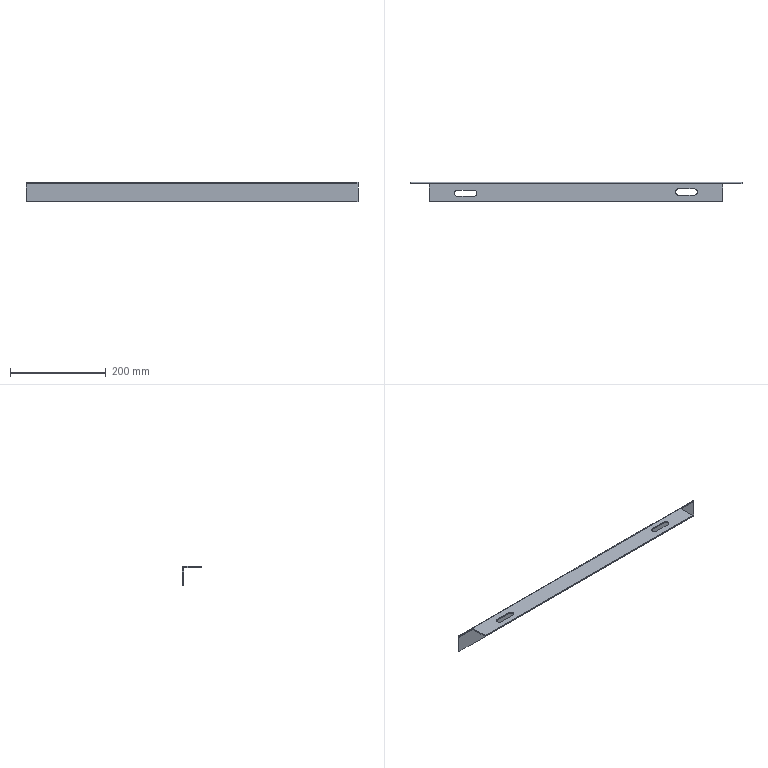Component | SolidWorks | BottomFrameAssembly2-1_CabinetWidthBeam-1 | 1 solid | 27 faces | box 695 x 40 x 40 mm | volume 123113 mm3 | plane 19 | cylinder 8 | commonest cylinder face diameters 13 x6 1 x1 6 x1
STEP:
#1=COLOUR_RGB('',0.7922,0.8196,0.9333);
#2=FILL_AREA_STYLE_COLOUR('',#1);
#3=FILL_AREA_STYLE('',(#2));
#4=SURFACE_STYLE_FILL_AREA(#3);
#5=SURFACE_SIDE_STYLE('',(#4));
#6=SURFACE_STYLE_USAGE(.BOTH.,#5);
#7=PRESENTATION_STYLE_ASSIGNMENT((#6));
#8=CARTESIAN_POINT('',(-1.991,5.157,66.928));
#9=VERTEX_POINT('',#8);
#10=CARTESIAN_POINT('',(-1.735,5.413,66.928));
#11=VERTEX_POINT('',#10);
#12=CARTESIAN_POINT('',(-1.735,5.157,66.928));
#13=DIRECTION('',(0.,-0.,-1.));
#14=DIRECTION('',(-1.,-0.,0.));
#15=AXIS2_PLACEMENT_3D('',#12,#13,#14);
#16=CIRCLE('',#15,0.2559);
#17=EDGE_CURVE('',#9,#11,#16,.T.);
#18=ORIENTED_EDGE('',*,*,#17,.F.);
#19=CARTESIAN_POINT('',(-1.991,5.157,66.83));
#20=VERTEX_POINT('',#19);
#21=CARTESIAN_POINT('',(-1.991,5.157,66.928));
#22=DIRECTION('',(0.,-0.,-1.));
#23=VECTOR('',#22,39.37);
#24=LINE('',#21,#23);
#25=EDGE_CURVE('',#9,#20,#24,.T.);
#26=ORIENTED_EDGE('',*,*,#25,.T.);
#27=CARTESIAN_POINT('',(-1.735,5.413,66.83));
#28=VERTEX_POINT('',#27);
#29=CARTESIAN_POINT('',(-1.735,5.157,66.83));
#30=DIRECTION('',(0.,-0.,-1.));
#31=DIRECTION('',(-1.,-0.,0.));
#32=AXIS2_PLACEMENT_3D('',#29,#30,#31);
#33=CIRCLE('',#32,0.2559);
#34=EDGE_CURVE('',#20,#28,#33,.T.);
#35=ORIENTED_EDGE('',*,*,#34,.T.);
#36=CARTESIAN_POINT('',(-1.735,5.413,66.928));
#37=DIRECTION('',(0.,-0.,-1.));
#38=VECTOR('',#37,39.37);
#39=LINE('',#36,#38);
#40=EDGE_CURVE('',#11,#28,#39,.T.);
#41=ORIENTED_EDGE('',*,*,#40,.F.);
#42=EDGE_LOOP('',(#18,#26,#35,#41));
#43=FACE_OUTER_BOUND('',#42,.T.);
#44=CARTESIAN_POINT('',(-1.735,5.157,66.928));
#45=DIRECTION('',(0.,-0.,-1.));
#46=DIRECTION('',(-1.,-0.,0.));
#47=AXIS2_PLACEMENT_3D('',#44,#45,#46);
#48=CYLINDRICAL_SURFACE('',#47,0.2559);
#49=ADVANCED_FACE('',(#43),#48,.F.);
#50=CARTESIAN_POINT('',(16.198,5.265,66.928));
#51=VERTEX_POINT('',#50);
#52=CARTESIAN_POINT('',(16.454,5.521,66.928));
#53=VERTEX_POINT('',#52);
#54=CARTESIAN_POINT('',(16.454,5.265,66.928));
#55=DIRECTION('',(0.,-0.,-1.));
#56=DIRECTION('',(-1.,-0.,0.));
#57=AXIS2_PLACEMENT_3D('',#54,#55,#56);
#58=CIRCLE('',#57,0.2559);
#59=EDGE_CURVE('',#51,#53,#58,.T.);
#60=ORIENTED_EDGE('',*,*,#59,.F.);
#61=CARTESIAN_POINT('',(16.198,5.265,66.83));
#62=VERTEX_POINT('',#61);
#63=CARTESIAN_POINT('',(16.198,5.265,66.928));
#64=DIRECTION('',(0.,-0.,-1.));
#65=VECTOR('',#64,39.37);
#66=LINE('',#63,#65);
#67=EDGE_CURVE('',#51,#62,#66,.T.);
#68=ORIENTED_EDGE('',*,*,#67,.T.);
#69=CARTESIAN_POINT('',(16.454,5.521,66.83));
#70=VERTEX_POINT('',#69);
#71=CARTESIAN_POINT('',(16.454,5.265,66.83));
#72=DIRECTION('',(0.,-0.,-1.));
#73=DIRECTION('',(-1.,-0.,0.));
#74=AXIS2_PLACEMENT_3D('',#71,#72,#73);
#75=CIRCLE('',#74,0.2559);
#76=EDGE_CURVE('',#62,#70,#75,.T.);
#77=ORIENTED_EDGE('',*,*,#76,.T.);
#78=CARTESIAN_POINT('',(16.454,5.521,66.928));
#79=DIRECTION('',(0.,-0.,-1.));
#80=VECTOR('',#79,39.37);
#81=LINE('',#78,#80);
#82=EDGE_CURVE('',#53,#70,#81,.T.);
#83=ORIENTED_EDGE('',*,*,#82,.F.);
#84=EDGE_LOOP('',(#60,#68,#77,#83));
#85=FACE_OUTER_BOUND('',#84,.T.);
#86=CARTESIAN_POINT('',(16.454,5.265,66.928));
#87=DIRECTION('',(0.,-0.,-1.));
#88=DIRECTION('',(-1.,-0.,0.));
#89=AXIS2_PLACEMENT_3D('',#86,#87,#88);
#90=CYLINDRICAL_SURFACE('',#89,0.2559);
#91=ADVANCED_FACE('',(#85),#90,.F.);
#92=CARTESIAN_POINT('',(-0.4356,5.413,66.83));
#93=VERTEX_POINT('',#92);
#94=CARTESIAN_POINT('',(-0.4356,4.901,66.83));
#95=VERTEX_POINT('',#94);
#96=CARTESIAN_POINT('',(-0.4356,5.157,66.83));
#97=DIRECTION('',(0.,-0.,-1.));
#98=DIRECTION('',(-1.,-0.,0.));
#99=AXIS2_PLACEMENT_3D('',#96,#97,#98);
#100=CIRCLE('',#99,0.2559);
#101=EDGE_CURVE('',#93,#95,#100,.T.);
#102=ORIENTED_EDGE('',*,*,#101,.F.);
#103=CARTESIAN_POINT('',(-0.4356,5.413,66.83));
#104=DIRECTION('',(1.,0.,-0.));
#105=VECTOR('',#104,39.37);
#106=LINE('',#103,#105);
#107=EDGE_CURVE('',#28,#93,#106,.T.);
#108=ORIENTED_EDGE('',*,*,#107,.F.);
#109=ORIENTED_EDGE('',*,*,#34,.F.);
#110=CARTESIAN_POINT('',(-1.735,4.901,66.83));
#111=VERTEX_POINT('',#110);
#112=CARTESIAN_POINT('',(-1.735,5.157,66.83));
#113=DIRECTION('',(0.,-0.,-1.));
#114=DIRECTION('',(-1.,-0.,0.));
#115=AXIS2_PLACEMENT_3D('',#112,#113,#114);
#116=CIRCLE('',#115,0.2559);
#117=EDGE_CURVE('',#111,#20,#116,.T.);
#118=ORIENTED_EDGE('',*,*,#117,.F.);
#119=CARTESIAN_POINT('',(-0.4356,4.901,66.83));
#120=DIRECTION('',(-1.,-0.,0.));
#121=VECTOR('',#120,39.37);
#122=LINE('',#119,#121);
#123=EDGE_CURVE('',#95,#111,#122,.T.);
#124=ORIENTED_EDGE('',*,*,#123,.F.);
#125=EDGE_LOOP('',(#102,#108,#109,#118,#124));
#126=FACE_BOUND('',#125,.T.);
#127=CARTESIAN_POINT('',(17.753,5.521,66.83));
#128=VERTEX_POINT('',#127);
#129=CARTESIAN_POINT('',(17.753,5.01,66.83));
#130=VERTEX_POINT('',#129);
#131=CARTESIAN_POINT('',(17.753,5.265,66.83));
#132=DIRECTION('',(0.,-0.,-1.));
#133=DIRECTION('',(-1.,-0.,0.));
#134=AXIS2_PLACEMENT_3D('',#131,#132,#133);
#135=CIRCLE('',#134,0.2559);
#136=EDGE_CURVE('',#128,#130,#135,.T.);
#137=ORIENTED_EDGE('',*,*,#136,.F.);
#138=CARTESIAN_POINT('',(17.753,5.521,66.83));
#139=DIRECTION('',(1.,0.,-0.));
#140=VECTOR('',#139,39.37);
#141=LINE('',#138,#140);
#142=EDGE_CURVE('',#70,#128,#141,.T.);
#143=ORIENTED_EDGE('',*,*,#142,.F.);
#144=ORIENTED_EDGE('',*,*,#76,.F.);
#145=CARTESIAN_POINT('',(16.454,5.01,66.83));
#146=VERTEX_POINT('',#145);
#147=CARTESIAN_POINT('',(16.454,5.265,66.83));
#148=DIRECTION('',(0.,-0.,-1.));
#149=DIRECTION('',(-1.,-0.,0.));
#150=AXIS2_PLACEMENT_3D('',#147,#148,#149);
#151=CIRCLE('',#150,0.2559);
#152=EDGE_CURVE('',#146,#62,#151,.T.);
#153=ORIENTED_EDGE('',*,*,#152,.F.);
#154=CARTESIAN_POINT('',(17.753,5.01,66.83));
#155=DIRECTION('',(-1.,-0.,0.));
#156=VECTOR('',#155,39.37);
#157=LINE('',#154,#156);
#158=EDGE_CURVE('',#130,#146,#157,.T.);
#159=ORIENTED_EDGE('',*,*,#158,.F.);
#160=EDGE_LOOP('',(#137,#143,#144,#153,#159));
#161=FACE_BOUND('',#160,.T.);
#162=CARTESIAN_POINT('',(-4.097,4.478,66.83));
#163=VERTEX_POINT('',#162);
#164=CARTESIAN_POINT('',(20.116,4.478,66.83));
#165=VERTEX_POINT('',#164);
#166=CARTESIAN_POINT('',(-5.672,4.478,66.83));
#167=DIRECTION('',(1.,0.,-0.));
#168=VECTOR('',#167,39.37);
#169=LINE('',#166,#168);
#170=EDGE_CURVE('',#163,#165,#169,.T.);
#171=ORIENTED_EDGE('',*,*,#170,.F.);
#172=CARTESIAN_POINT('',(-4.097,5.935,66.83));
#173=VERTEX_POINT('',#172);
#174=CARTESIAN_POINT('',(-4.097,5.935,66.83));
#175=DIRECTION('',(0.,-1.,0.));
#176=VECTOR('',#175,39.37);
#177=LINE('',#174,#176);
#178=EDGE_CURVE('',#173,#163,#177,.T.);
#179=ORIENTED_EDGE('',*,*,#178,.F.);
#180=CARTESIAN_POINT('',(20.116,5.935,66.83));
#181=VERTEX_POINT('',#180);
#182=CARTESIAN_POINT('',(-5.672,5.935,66.83));
#183=DIRECTION('',(1.,0.,-0.));
#184=VECTOR('',#183,39.37);
#185=LINE('',#182,#184);
#186=EDGE_CURVE('',#173,#181,#185,.T.);
#187=ORIENTED_EDGE('',*,*,#186,.T.);
#188=CARTESIAN_POINT('',(20.116,4.478,66.83));
#189=DIRECTION('',(-0.,1.,-0.));
#190=VECTOR('',#189,39.37);
#191=LINE('',#188,#190);
#192=EDGE_CURVE('',#165,#181,#191,.T.);
#193=ORIENTED_EDGE('',*,*,#192,.F.);
#194=EDGE_LOOP('',(#171,#179,#187,#193));
#195=FACE_OUTER_BOUND('',#194,.T.);
#196=CARTESIAN_POINT('',(-5.672,4.478,66.83));
#197=DIRECTION('',(0.,-0.,-1.));
#198=DIRECTION('',(-1.,-0.,0.));
#199=AXIS2_PLACEMENT_3D('',#196,#197,#198);
#200=PLANE('',#199);
#201=ADVANCED_FACE('',(#126,#161,#195),#200,.T.);
#202=CARTESIAN_POINT('',(-4.097,4.478,66.928));
#203=VERTEX_POINT('',#202);
#204=CARTESIAN_POINT('',(20.116,4.478,66.928));
#205=VERTEX_POINT('',#204);
#206=CARTESIAN_POINT('',(-5.672,4.478,66.928));
#207=DIRECTION('',(1.,0.,-0.));
#208=VECTOR('',#207,39.37);
#209=LINE('',#206,#208);
#210=EDGE_CURVE('',#203,#205,#209,.T.);
#211=ORIENTED_EDGE('',*,*,#210,.F.);
#212=CARTESIAN_POINT('',(-4.097,4.478,66.83));
#213=DIRECTION('',(0.,0.,1.));
#214=VECTOR('',#213,39.37);
#215=LINE('',#212,#214);
#216=EDGE_CURVE('',#163,#203,#215,.T.);
#217=ORIENTED_EDGE('',*,*,#216,.F.);
#218=ORIENTED_EDGE('',*,*,#170,.T.);
#219=CARTESIAN_POINT('',(20.116,4.478,66.928));
#220=DIRECTION('',(0.,-0.,-1.));
#221=VECTOR('',#220,39.37);
#222=LINE('',#219,#221);
#223=EDGE_CURVE('',#205,#165,#222,.T.);
#224=ORIENTED_EDGE('',*,*,#223,.F.);
#225=EDGE_LOOP('',(#211,#217,#218,#224));
#226=FACE_OUTER_BOUND('',#225,.T.);
#227=CARTESIAN_POINT('',(-5.672,4.478,66.928));
#228=DIRECTION('',(0.,-1.,0.));
#229=DIRECTION('',(-1.,-0.,0.));
#230=AXIS2_PLACEMENT_3D('',#227,#228,#229);
#231=PLANE('',#230);
#232=ADVANCED_FACE('',(#226),#231,.T.);
#233=CARTESIAN_POINT('',(-0.4356,5.413,66.928));
#234=VERTEX_POINT('',#233);
#235=CARTESIAN_POINT('',(-0.4356,5.413,66.928));
#236=DIRECTION('',(1.,0.,-0.));
#237=VECTOR('',#236,39.37);
#238=LINE('',#235,#237);
#239=EDGE_CURVE('',#11,#234,#238,.T.);
#240=ORIENTED_EDGE('',*,*,#239,.T.);
#241=CARTESIAN_POINT('',(-0.4356,4.901,66.928));
#242=VERTEX_POINT('',#241);
#243=CARTESIAN_POINT('',(-0.4356,5.157,66.928));
#244=DIRECTION('',(0.,-0.,-1.));
#245=DIRECTION('',(-1.,-0.,0.));
#246=AXIS2_PLACEMENT_3D('',#243,#244,#245);
#247=CIRCLE('',#246,0.2559);
#248=EDGE_CURVE('',#234,#242,#247,.T.);
#249=ORIENTED_EDGE('',*,*,#248,.T.);
#250=CARTESIAN_POINT('',(-1.735,4.901,66.928));
#251=VERTEX_POINT('',#250);
#252=CARTESIAN_POINT('',(-0.4356,4.901,66.928));
#253=DIRECTION('',(-1.,-0.,0.));
#254=VECTOR('',#253,39.37);
#255=LINE('',#252,#254);
#256=EDGE_CURVE('',#242,#251,#255,.T.);
#257=ORIENTED_EDGE('',*,*,#256,.T.);
#258=CARTESIAN_POINT('',(-1.735,5.157,66.928));
#259=DIRECTION('',(0.,-0.,-1.));
#260=DIRECTION('',(-1.,-0.,0.));
#261=AXIS2_PLACEMENT_3D('',#258,#259,#260);
#262=CIRCLE('',#261,0.2559);
#263=EDGE_CURVE('',#251,#9,#262,.T.);
#264=ORIENTED_EDGE('',*,*,#263,.T.);
#265=ORIENTED_EDGE('',*,*,#17,.T.);
#266=EDGE_LOOP('',(#240,#249,#257,#264,#265));
#267=FACE_BOUND('',#266,.T.);
#268=CARTESIAN_POINT('',(17.753,5.521,66.928));
#269=VERTEX_POINT('',#268);
#270=CARTESIAN_POINT('',(17.753,5.521,66.928));
#271=DIRECTION('',(1.,0.,-0.));
#272=VECTOR('',#271,39.37);
#273=LINE('',#270,#272);
#274=EDGE_CURVE('',#53,#269,#273,.T.);
#275=ORIENTED_EDGE('',*,*,#274,.T.);
#276=CARTESIAN_POINT('',(17.753,5.01,66.928));
#277=VERTEX_POINT('',#276);
#278=CARTESIAN_POINT('',(17.753,5.265,66.928));
#279=DIRECTION('',(0.,-0.,-1.));
#280=DIRECTION('',(-1.,-0.,0.));
#281=AXIS2_PLACEMENT_3D('',#278,#279,#280);
#282=CIRCLE('',#281,0.2559);
#283=EDGE_CURVE('',#269,#277,#282,.T.);
#284=ORIENTED_EDGE('',*,*,#283,.T.);
#285=CARTESIAN_POINT('',(16.454,5.01,66.928));
#286=VERTEX_POINT('',#285);
#287=CARTESIAN_POINT('',(17.753,5.01,66.928));
#288=DIRECTION('',(-1.,-0.,0.));
#289=VECTOR('',#288,39.37);
#290=LINE('',#287,#289);
#291=EDGE_CURVE('',#277,#286,#290,.T.);
#292=ORIENTED_EDGE('',*,*,#291,.T.);
#293=CARTESIAN_POINT('',(16.454,5.265,66.928));
#294=DIRECTION('',(0.,-0.,-1.));
#295=DIRECTION('',(-1.,-0.,0.));
#296=AXIS2_PLACEMENT_3D('',#293,#294,#295);
#297=CIRCLE('',#296,0.2559);
#298=EDGE_CURVE('',#286,#51,#297,.T.);
#299=ORIENTED_EDGE('',*,*,#298,.T.);
#300=ORIENTED_EDGE('',*,*,#59,.T.);
#301=EDGE_LOOP('',(#275,#284,#292,#299,#300));
#302=FACE_BOUND('',#301,.T.);
#303=CARTESIAN_POINT('',(-4.097,5.935,66.928));
#304=VERTEX_POINT('',#303);
#305=CARTESIAN_POINT('',(-4.097,4.478,66.928));
#306=DIRECTION('',(0.,-1.,0.));
#307=VECTOR('',#306,39.37);
#308=LINE('',#305,#307);
#309=EDGE_CURVE('',#304,#203,#308,.T.);
#310=ORIENTED_EDGE('',*,*,#309,.T.);
#311=ORIENTED_EDGE('',*,*,#210,.T.);
#312=CARTESIAN_POINT('',(20.116,5.935,66.928));
#313=VERTEX_POINT('',#312);
#314=CARTESIAN_POINT('',(20.116,4.478,66.928));
#315=DIRECTION('',(-0.,1.,-0.));
#316=VECTOR('',#315,39.37);
#317=LINE('',#314,#316);
#318=EDGE_CURVE('',#205,#313,#317,.T.);
#319=ORIENTED_EDGE('',*,*,#318,.T.);
#320=CARTESIAN_POINT('',(-5.672,5.935,66.928));
#321=DIRECTION('',(1.,0.,-0.));
#322=VECTOR('',#321,39.37);
#323=LINE('',#320,#322);
#324=EDGE_CURVE('',#304,#313,#323,.T.);
#325=ORIENTED_EDGE('',*,*,#324,.F.);
#326=EDGE_LOOP('',(#310,#311,#319,#325));
#327=FACE_OUTER_BOUND('',#326,.T.);
#328=CARTESIAN_POINT('',(-5.672,4.478,66.928));
#329=DIRECTION('',(0.,-0.,-1.));
#330=DIRECTION('',(-1.,-0.,0.));
#331=AXIS2_PLACEMENT_3D('',#328,#329,#330);
#332=PLANE('',#331);
#333=ADVANCED_FACE('',(#267,#302,#327),#332,.F.);
#334=CARTESIAN_POINT('',(21.69,5.954,66.927));
#335=VERTEX_POINT('',#334);
#336=CARTESIAN_POINT('',(21.69,6.053,66.81));
#337=VERTEX_POINT('',#336);
#338=CARTESIAN_POINT('',(21.69,5.935,66.81));
#339=DIRECTION('',(-1.,-0.,0.));
#340=DIRECTION('',(0.,1.,0.));
#341=AXIS2_PLACEMENT_3D('',#338,#339,#340);
#342=CIRCLE('',#341,0.1181);
#343=EDGE_CURVE('',#335,#337,#342,.T.);
#344=ORIENTED_EDGE('',*,*,#343,.F.);
#345=CARTESIAN_POINT('',(21.69,5.938,66.83));
#346=VERTEX_POINT('',#345);
#347=CARTESIAN_POINT('',(21.69,5.954,66.927));
#348=DIRECTION('',(0.,-0.1667,-0.986));
#349=VECTOR('',#348,39.37);
#350=LINE('',#347,#349);
#351=EDGE_CURVE('',#335,#346,#350,.T.);
#352=ORIENTED_EDGE('',*,*,#351,.T.);
#353=CARTESIAN_POINT('',(21.69,5.954,66.81));
#354=VERTEX_POINT('',#353);
#355=CARTESIAN_POINT('',(21.69,5.935,66.81));
#356=DIRECTION('',(-1.,-0.,0.));
#357=DIRECTION('',(0.,-1.,0.));
#358=AXIS2_PLACEMENT_3D('',#355,#356,#357);
#359=CIRCLE('',#358,0.01969);
#360=EDGE_CURVE('',#346,#354,#359,.T.);
#361=ORIENTED_EDGE('',*,*,#360,.T.);
#362=CARTESIAN_POINT('',(21.69,6.053,66.81));
#363=DIRECTION('',(0.,-1.,0.));
#364=VECTOR('',#363,39.37);
#365=LINE('',#362,#364);
#366=EDGE_CURVE('',#337,#354,#365,.T.);
#367=ORIENTED_EDGE('',*,*,#366,.F.);
#368=EDGE_LOOP('',(#344,#352,#361,#367));
#369=FACE_OUTER_BOUND('',#368,.T.);
#370=CARTESIAN_POINT('',(21.69,5.935,66.83));
#371=DIRECTION('',(1.,0.,-0.));
#372=DIRECTION('',(0.,-1.,0.));
#373=AXIS2_PLACEMENT_3D('',#370,#371,#372);
#374=PLANE('',#373);
#375=ADVANCED_FACE('',(#369),#374,.T.);
#376=ORIENTED_EDGE('',*,*,#360,.F.);
#377=CARTESIAN_POINT('',(20.116,5.938,66.83));
#378=VERTEX_POINT('',#377);
#379=CARTESIAN_POINT('',(-5.672,5.938,66.83));
#380=DIRECTION('',(1.,0.,-0.));
#381=VECTOR('',#380,39.37);
#382=LINE('',#379,#381);
#383=EDGE_CURVE('',#378,#346,#382,.T.);
#384=ORIENTED_EDGE('',*,*,#383,.F.);
#385=CARTESIAN_POINT('',(20.116,5.935,66.81));
#386=DIRECTION('',(-1.,-0.,0.));
#387=DIRECTION('',(0.,-1.,0.));
#388=AXIS2_PLACEMENT_3D('',#385,#386,#387);
#389=CIRCLE('',#388,0.01969);
#390=EDGE_CURVE('',#181,#378,#389,.T.);
#391=ORIENTED_EDGE('',*,*,#390,.F.);
#392=ORIENTED_EDGE('',*,*,#186,.F.);
#393=CARTESIAN_POINT('',(-5.672,5.935,66.83));
#394=VERTEX_POINT('',#393);
#395=CARTESIAN_POINT('',(-5.672,5.935,66.83));
#396=DIRECTION('',(1.,0.,-0.));
#397=VECTOR('',#396,39.37);
#398=LINE('',#395,#397);
#399=EDGE_CURVE('',#394,#173,#398,.T.);
#400=ORIENTED_EDGE('',*,*,#399,.F.);
#401=CARTESIAN_POINT('',(-5.672,5.954,66.81));
#402=VERTEX_POINT('',#401);
#403=CARTESIAN_POINT('',(-5.672,5.935,66.81));
#404=DIRECTION('',(-1.,-0.,0.));
#405=DIRECTION('',(0.,-1.,0.));
#406=AXIS2_PLACEMENT_3D('',#403,#404,#405);
#407=CIRCLE('',#406,0.01969);
#408=EDGE_CURVE('',#394,#402,#407,.T.);
#409=ORIENTED_EDGE('',*,*,#408,.T.);
#410=CARTESIAN_POINT('',(-5.672,5.954,66.81));
#411=DIRECTION('',(1.,0.,-0.));
#412=VECTOR('',#411,39.37);
#413=LINE('',#410,#412);
#414=EDGE_CURVE('',#402,#354,#413,.T.);
#415=ORIENTED_EDGE('',*,*,#414,.T.);
#416=EDGE_LOOP('',(#376,#384,#391,#392,#400,#409,#415));
#417=FACE_OUTER_BOUND('',#416,.T.);
#418=CARTESIAN_POINT('',(-5.672,5.935,66.81));
#419=DIRECTION('',(1.,0.,-0.));
#420=DIRECTION('',(0.,-1.,0.));
#421=AXIS2_PLACEMENT_3D('',#418,#419,#420);
#422=CYLINDRICAL_SURFACE('',#421,0.01969);
#423=ADVANCED_FACE('',(#417),#422,.F.);
#424=CARTESIAN_POINT('',(20.116,5.954,66.927));
#425=VERTEX_POINT('',#424);
#426=CARTESIAN_POINT('',(-5.672,5.954,66.927));
#427=DIRECTION('',(1.,0.,-0.));
#428=VECTOR('',#427,39.37);
#429=LINE('',#426,#428);
#430=EDGE_CURVE('',#425,#335,#429,.T.);
#431=ORIENTED_EDGE('',*,*,#430,.T.);
#432=ORIENTED_EDGE('',*,*,#343,.T.);
#433=CARTESIAN_POINT('',(-5.672,6.053,66.81));
#434=VERTEX_POINT('',#433);
#435=CARTESIAN_POINT('',(-5.672,6.053,66.81));
#436=DIRECTION('',(1.,0.,-0.));
#437=VECTOR('',#436,39.37);
#438=LINE('',#435,#437);
#439=EDGE_CURVE('',#434,#337,#438,.T.);
#440=ORIENTED_EDGE('',*,*,#439,.F.);
#441=CARTESIAN_POINT('',(-5.672,5.935,66.928));
#442=VERTEX_POINT('',#441);
#443=CARTESIAN_POINT('',(-5.672,5.935,66.81));
#444=DIRECTION('',(-1.,-0.,0.));
#445=DIRECTION('',(-0.,1.,0.));
#446=AXIS2_PLACEMENT_3D('',#443,#444,#445);
#447=CIRCLE('',#446,0.1181);
#448=EDGE_CURVE('',#442,#434,#447,.T.);
#449=ORIENTED_EDGE('',*,*,#448,.F.);
#450=CARTESIAN_POINT('',(-5.672,5.935,66.928));
#451=DIRECTION('',(1.,0.,-0.));
#452=VECTOR('',#451,39.37);
#453=LINE('',#450,#452);
#454=EDGE_CURVE('',#442,#304,#453,.T.);
#455=ORIENTED_EDGE('',*,*,#454,.T.);
#456=ORIENTED_EDGE('',*,*,#324,.T.);
#457=CARTESIAN_POINT('',(20.116,5.935,66.81));
#458=DIRECTION('',(-1.,-0.,0.));
#459=DIRECTION('',(0.,1.,0.));
#460=AXIS2_PLACEMENT_3D('',#457,#458,#459);
#461=CIRCLE('',#460,0.1181);
#462=EDGE_CURVE('',#313,#425,#461,.T.);
#463=ORIENTED_EDGE('',*,*,#462,.T.);
#464=EDGE_LOOP('',(#431,#432,#440,#449,#455,#456,#463));
#465=FACE_OUTER_BOUND('',#464,.T.);
#466=CARTESIAN_POINT('',(-5.672,5.935,66.81));
#467=DIRECTION('',(1.,0.,-0.));
#468=DIRECTION('',(0.,-1.,0.));
#469=AXIS2_PLACEMENT_3D('',#466,#467,#468);
#470=CYLINDRICAL_SURFACE('',#469,0.1181);
#471=ADVANCED_FACE('',(#465),#470,.T.);
#472=CARTESIAN_POINT('',(-5.672,5.954,66.81));
#473=DIRECTION('',(-0.,1.,-0.));
#474=VECTOR('',#473,39.37);
#475=LINE('',#472,#474);
#476=EDGE_CURVE('',#402,#434,#475,.T.);
#477=ORIENTED_EDGE('',*,*,#476,.F.);
#478=ORIENTED_EDGE('',*,*,#408,.F.);
#479=CARTESIAN_POINT('',(-5.672,5.935,66.928));
#480=DIRECTION('',(0.,-0.,-1.));
#481=VECTOR('',#480,39.37);
#482=LINE('',#479,#481);
#483=EDGE_CURVE('',#442,#394,#482,.T.);
#484=ORIENTED_EDGE('',*,*,#483,.F.);
#485=ORIENTED_EDGE('',*,*,#448,.T.);
#486=EDGE_LOOP('',(#477,#478,#484,#485));
#487=FACE_OUTER_BOUND('',#486,.T.);
#488=CARTESIAN_POINT('',(-5.672,5.954,66.81));
#489=DIRECTION('',(-1.,-0.,0.));
#490=DIRECTION('',(-0.,1.,-0.));
#491=AXIS2_PLACEMENT_3D('',#488,#489,#490);
#492=PLANE('',#491);
#493=ADVANCED_FACE('',(#487),#492,.T.);
#494=CARTESIAN_POINT('',(-5.672,5.954,65.354));
#495=VERTEX_POINT('',#494);
#496=CARTESIAN_POINT('',(-5.672,5.954,66.83));
#497=DIRECTION('',(0.,-0.,-1.));
#498=VECTOR('',#497,39.37);
#499=LINE('',#496,#498);
#500=EDGE_CURVE('',#402,#495,#499,.T.);
#501=ORIENTED_EDGE('',*,*,#500,.F.);
#502=ORIENTED_EDGE('',*,*,#476,.T.);
#503=CARTESIAN_POINT('',(-5.672,6.053,65.354));
#504=VERTEX_POINT('',#503);
#505=CARTESIAN_POINT('',(-5.672,6.053,66.83));
#506=DIRECTION('',(0.,-0.,-1.));
#507=VECTOR('',#506,39.37);
#508=LINE('',#505,#507);
#509=EDGE_CURVE('',#434,#504,#508,.T.);
#510=ORIENTED_EDGE('',*,*,#509,.T.);
#511=CARTESIAN_POINT('',(-5.672,5.954,65.354));
#512=DIRECTION('',(-0.,1.,-0.));
#513=VECTOR('',#512,39.37);
#514=LINE('',#511,#513);
#515=EDGE_CURVE('',#495,#504,#514,.T.);
#516=ORIENTED_EDGE('',*,*,#515,.F.);
#517=EDGE_LOOP('',(#501,#502,#510,#516));
#518=FACE_OUTER_BOUND('',#517,.T.);
#519=CARTESIAN_POINT('',(-5.672,5.935,66.928));
#520=DIRECTION('',(-1.,-0.,0.));
#521=DIRECTION('',(-0.,1.,-0.));
#522=AXIS2_PLACEMENT_3D('',#519,#520,#521);
#523=PLANE('',#522);
#524=ADVANCED_FACE('',(#518),#523,.T.);
#525=CARTESIAN_POINT('',(21.69,6.053,65.354));
#526=VERTEX_POINT('',#525);
#527=CARTESIAN_POINT('',(21.69,6.053,66.83));
#528=DIRECTION('',(0.,-0.,-1.));
#529=VECTOR('',#528,39.37);
#530=LINE('',#527,#529);
#531=EDGE_CURVE('',#337,#526,#530,.T.);
#532=ORIENTED_EDGE('',*,*,#531,.T.);
#533=CARTESIAN_POINT('',(-5.672,6.053,65.354));
#534=DIRECTION('',(1.,0.,-0.));
#535=VECTOR('',#534,39.37);
#536=LINE('',#533,#535);
#537=EDGE_CURVE('',#504,#526,#536,.T.);
#538=ORIENTED_EDGE('',*,*,#537,.F.);
#539=ORIENTED_EDGE('',*,*,#509,.F.);
#540=ORIENTED_EDGE('',*,*,#439,.T.);
#541=EDGE_LOOP('',(#532,#538,#539,#540));
#542=FACE_OUTER_BOUND('',#541,.T.);
#543=CARTESIAN_POINT('',(-5.672,6.053,66.83));
#544=DIRECTION('',(0.,-1.,0.));
#545=DIRECTION('',(-1.,-0.,0.));
#546=AXIS2_PLACEMENT_3D('',#543,#544,#545);
#547=PLANE('',#546);
#548=ADVANCED_FACE('',(#542),#547,.F.);
#549=CARTESIAN_POINT('',(21.69,5.954,65.354));
#550=VERTEX_POINT('',#549);
#551=CARTESIAN_POINT('',(21.69,5.954,65.354));
#552=DIRECTION('',(-0.,1.,-0.));
#553=VECTOR('',#552,39.37);
#554=LINE('',#551,#553);
#555=EDGE_CURVE('',#550,#526,#554,.T.);
#556=ORIENTED_EDGE('',*,*,#555,.F.);
#557=CARTESIAN_POINT('',(-5.672,5.954,65.354));
#558=DIRECTION('',(1.,0.,-0.));
#559=VECTOR('',#558,39.37);
#560=LINE('',#557,#559);
#561=EDGE_CURVE('',#495,#550,#560,.T.);
#562=ORIENTED_EDGE('',*,*,#561,.F.);
#563=ORIENTED_EDGE('',*,*,#515,.T.);
#564=ORIENTED_EDGE('',*,*,#537,.T.);
#565=EDGE_LOOP('',(#556,#562,#563,#564));
#566=FACE_OUTER_BOUND('',#565,.T.);
#567=CARTESIAN_POINT('',(-5.672,5.954,65.354));
#568=DIRECTION('',(0.,-0.,-1.));
#569=DIRECTION('',(-1.,-0.,0.));
#570=AXIS2_PLACEMENT_3D('',#567,#568,#569);
#571=PLANE('',#570);
#572=ADVANCED_FACE('',(#566),#571,.T.);
#573=CARTESIAN_POINT('',(21.69,5.954,66.83));
#574=DIRECTION('',(0.,-0.,-1.));
#575=VECTOR('',#574,39.37);
#576=LINE('',#573,#575);
#577=EDGE_CURVE('',#354,#550,#576,.T.);
#578=ORIENTED_EDGE('',*,*,#577,.F.);
#579=ORIENTED_EDGE('',*,*,#414,.F.);
#580=ORIENTED_EDGE('',*,*,#500,.T.);
#581=ORIENTED_EDGE('',*,*,#561,.T.);
#582=EDGE_LOOP('',(#578,#579,#580,#581));
#583=FACE_OUTER_BOUND('',#582,.T.);
#584=CARTESIAN_POINT('',(-5.672,5.954,66.83));
#585=DIRECTION('',(0.,-1.,0.));
#586=DIRECTION('',(-1.,-0.,0.));
#587=AXIS2_PLACEMENT_3D('',#584,#585,#586);
#588=PLANE('',#587);
#589=ADVANCED_FACE('',(#583),#588,.T.);
#590=ORIENTED_EDGE('',*,*,#531,.F.);
#591=ORIENTED_EDGE('',*,*,#366,.T.);
#592=ORIENTED_EDGE('',*,*,#577,.T.);
#593=ORIENTED_EDGE('',*,*,#555,.T.);
#594=EDGE_LOOP('',(#590,#591,#592,#593));
#595=FACE_OUTER_BOUND('',#594,.T.);
#596=CARTESIAN_POINT('',(21.69,5.935,66.81));
#597=DIRECTION('',(1.,0.,-0.));
#598=DIRECTION('',(0.,-1.,0.));
#599=AXIS2_PLACEMENT_3D('',#596,#597,#598);
#600=PLANE('',#599);
#601=ADVANCED_FACE('',(#595),#600,.T.);
#602=ORIENTED_EDGE('',*,*,#136,.T.);
#603=CARTESIAN_POINT('',(17.753,5.01,66.928));
#604=DIRECTION('',(0.,-0.,-1.));
#605=VECTOR('',#604,39.37);
#606=LINE('',#603,#605);
#607=EDGE_CURVE('',#277,#130,#606,.T.);
#608=ORIENTED_EDGE('',*,*,#607,.F.);
#609=ORIENTED_EDGE('',*,*,#283,.F.);
#610=CARTESIAN_POINT('',(17.753,5.521,66.928));
#611=DIRECTION('',(0.,-0.,-1.));
#612=VECTOR('',#611,39.37);
#613=LINE('',#610,#612);
#614=EDGE_CURVE('',#269,#128,#613,.T.);
#615=ORIENTED_EDGE('',*,*,#614,.T.);
#616=EDGE_LOOP('',(#602,#608,#609,#615));
#617=FACE_OUTER_BOUND('',#616,.T.);
#618=CARTESIAN_POINT('',(17.753,5.265,66.928));
#619=DIRECTION('',(0.,-0.,-1.));
#620=DIRECTION('',(-1.,-0.,0.));
#621=AXIS2_PLACEMENT_3D('',#618,#619,#620);
#622=CYLINDRICAL_SURFACE('',#621,0.2559);
#623=ADVANCED_FACE('',(#617),#622,.F.);
#624=ORIENTED_EDGE('',*,*,#142,.T.);
#625=ORIENTED_EDGE('',*,*,#614,.F.);
#626=ORIENTED_EDGE('',*,*,#274,.F.);
#627=ORIENTED_EDGE('',*,*,#82,.T.);
#628=EDGE_LOOP('',(#624,#625,#626,#627));
#629=FACE_OUTER_BOUND('',#628,.T.);
#630=CARTESIAN_POINT('',(17.753,5.521,66.928));
#631=DIRECTION('',(-0.,1.,-0.));
#632=DIRECTION('',(1.,0.,-0.));
#633=AXIS2_PLACEMENT_3D('',#630,#631,#632);
#634=PLANE('',#633);
#635=ADVANCED_FACE('',(#629),#634,.F.);
#636=ORIENTED_EDGE('',*,*,#67,.F.);
#637=ORIENTED_EDGE('',*,*,#298,.F.);
#638=CARTESIAN_POINT('',(16.454,5.01,66.928));
#639=DIRECTION('',(0.,-0.,-1.));
#640=VECTOR('',#639,39.37);
#641=LINE('',#638,#640);
#642=EDGE_CURVE('',#286,#146,#641,.T.);
#643=ORIENTED_EDGE('',*,*,#642,.T.);
#644=ORIENTED_EDGE('',*,*,#152,.T.);
#645=EDGE_LOOP('',(#636,#637,#643,#644));
#646=FACE_OUTER_BOUND('',#645,.T.);
#647=CARTESIAN_POINT('',(16.454,5.265,66.928));
#648=DIRECTION('',(0.,-0.,-1.));
#649=DIRECTION('',(-1.,-0.,0.));
#650=AXIS2_PLACEMENT_3D('',#647,#648,#649);
#651=CYLINDRICAL_SURFACE('',#650,0.2559);
#652=ADVANCED_FACE('',(#646),#651,.F.);
#653=ORIENTED_EDGE('',*,*,#158,.T.);
#654=ORIENTED_EDGE('',*,*,#642,.F.);
#655=ORIENTED_EDGE('',*,*,#291,.F.);
#656=ORIENTED_EDGE('',*,*,#607,.T.);
#657=EDGE_LOOP('',(#653,#654,#655,#656));
#658=FACE_OUTER_BOUND('',#657,.T.);
#659=CARTESIAN_POINT('',(17.753,5.01,66.928));
#660=DIRECTION('',(0.,-1.,0.));
#661=DIRECTION('',(-1.,-0.,0.));
#662=AXIS2_PLACEMENT_3D('',#659,#660,#661);
#663=PLANE('',#662);
#664=ADVANCED_FACE('',(#658),#663,.F.);
#665=ORIENTED_EDGE('',*,*,#101,.T.);
#666=CARTESIAN_POINT('',(-0.4356,4.901,66.928));
#667=DIRECTION('',(0.,-0.,-1.));
#668=VECTOR('',#667,39.37);
#669=LINE('',#666,#668);
#670=EDGE_CURVE('',#242,#95,#669,.T.);
#671=ORIENTED_EDGE('',*,*,#670,.F.);
#672=ORIENTED_EDGE('',*,*,#248,.F.);
#673=CARTESIAN_POINT('',(-0.4356,5.413,66.928));
#674=DIRECTION('',(0.,-0.,-1.));
#675=VECTOR('',#674,39.37);
#676=LINE('',#673,#675);
#677=EDGE_CURVE('',#234,#93,#676,.T.);
#678=ORIENTED_EDGE('',*,*,#677,.T.);
#679=EDGE_LOOP('',(#665,#671,#672,#678));
#680=FACE_OUTER_BOUND('',#679,.T.);
#681=CARTESIAN_POINT('',(-0.4356,5.157,66.928));
#682=DIRECTION('',(0.,-0.,-1.));
#683=DIRECTION('',(-1.,-0.,0.));
#684=AXIS2_PLACEMENT_3D('',#681,#682,#683);
#685=CYLINDRICAL_SURFACE('',#684,0.2559);
#686=ADVANCED_FACE('',(#680),#685,.F.);
#687=ORIENTED_EDGE('',*,*,#107,.T.);
#688=ORIENTED_EDGE('',*,*,#677,.F.);
#689=ORIENTED_EDGE('',*,*,#239,.F.);
#690=ORIENTED_EDGE('',*,*,#40,.T.);
#691=EDGE_LOOP('',(#687,#688,#689,#690));
#692=FACE_OUTER_BOUND('',#691,.T.);
#693=CARTESIAN_POINT('',(-0.4356,5.413,66.928));
#694=DIRECTION('',(-0.,1.,-0.));
#695=DIRECTION('',(1.,0.,-0.));
#696=AXIS2_PLACEMENT_3D('',#693,#694,#695);
#697=PLANE('',#696);
#698=ADVANCED_FACE('',(#692),#697,.F.);
#699=ORIENTED_EDGE('',*,*,#25,.F.);
#700=ORIENTED_EDGE('',*,*,#263,.F.);
#701=CARTESIAN_POINT('',(-1.735,4.901,66.928));
#702=DIRECTION('',(0.,-0.,-1.));
#703=VECTOR('',#702,39.37);
#704=LINE('',#701,#703);
#705=EDGE_CURVE('',#251,#111,#704,.T.);
#706=ORIENTED_EDGE('',*,*,#705,.T.);
#707=ORIENTED_EDGE('',*,*,#117,.T.);
#708=EDGE_LOOP('',(#699,#700,#706,#707));
#709=FACE_OUTER_BOUND('',#708,.T.);
#710=CARTESIAN_POINT('',(-1.735,5.157,66.928));
#711=DIRECTION('',(0.,-0.,-1.));
#712=DIRECTION('',(-1.,-0.,0.));
#713=AXIS2_PLACEMENT_3D('',#710,#711,#712);
#714=CYLINDRICAL_SURFACE('',#713,0.2559);
#715=ADVANCED_FACE('',(#709),#714,.F.);
#716=ORIENTED_EDGE('',*,*,#123,.T.);
#717=ORIENTED_EDGE('',*,*,#705,.F.);
#718=ORIENTED_EDGE('',*,*,#256,.F.);
#719=ORIENTED_EDGE('',*,*,#670,.T.);
#720=EDGE_LOOP('',(#716,#717,#718,#719));
#721=FACE_OUTER_BOUND('',#720,.T.);
#722=CARTESIAN_POINT('',(-0.4356,4.901,66.928));
#723=DIRECTION('',(0.,-1.,0.));
#724=DIRECTION('',(-1.,-0.,0.));
#725=AXIS2_PLACEMENT_3D('',#722,#723,#724);
#726=PLANE('',#725);
#727=ADVANCED_FACE('',(#721),#726,.F.);
#728=CARTESIAN_POINT('',(20.116,5.935,66.928));
#729=DIRECTION('',(0.,-0.,-1.));
#730=VECTOR('',#729,39.37);
#731=LINE('',#728,#730);
#732=EDGE_CURVE('',#313,#181,#731,.T.);
#733=ORIENTED_EDGE('',*,*,#732,.F.);
#734=ORIENTED_EDGE('',*,*,#318,.F.);
#735=ORIENTED_EDGE('',*,*,#223,.T.);
#736=ORIENTED_EDGE('',*,*,#192,.T.);
#737=EDGE_LOOP('',(#733,#734,#735,#736));
#738=FACE_OUTER_BOUND('',#737,.T.);
#739=CARTESIAN_POINT('',(20.116,4.478,66.928));
#740=DIRECTION('',(-1.,-0.,0.));
#741=DIRECTION('',(-0.,1.,-0.));
#742=AXIS2_PLACEMENT_3D('',#739,#740,#741);
#743=PLANE('',#742);
#744=ADVANCED_FACE('',(#738),#743,.F.);
#745=ORIENTED_EDGE('',*,*,#351,.F.);
#746=ORIENTED_EDGE('',*,*,#430,.F.);
#747=CARTESIAN_POINT('',(20.116,5.954,66.927));
#748=DIRECTION('',(0.,-0.1667,-0.986));
#749=VECTOR('',#748,39.37);
#750=LINE('',#747,#749);
#751=EDGE_CURVE('',#425,#378,#750,.T.);
#752=ORIENTED_EDGE('',*,*,#751,.T.);
#753=ORIENTED_EDGE('',*,*,#383,.T.);
#754=EDGE_LOOP('',(#745,#746,#752,#753));
#755=FACE_OUTER_BOUND('',#754,.T.);
#756=CARTESIAN_POINT('',(20.903,5.954,66.927));
#757=DIRECTION('',(0.,-0.986,0.1667));
#758=DIRECTION('',(1.,0.,-0.));
#759=AXIS2_PLACEMENT_3D('',#756,#757,#758);
#760=PLANE('',#759);
#761=ADVANCED_FACE('',(#755),#760,.T.);
#762=ORIENTED_EDGE('',*,*,#462,.F.);
#763=ORIENTED_EDGE('',*,*,#732,.T.);
#764=ORIENTED_EDGE('',*,*,#390,.T.);
#765=ORIENTED_EDGE('',*,*,#751,.F.);
#766=EDGE_LOOP('',(#762,#763,#764,#765));
#767=FACE_OUTER_BOUND('',#766,.T.);
#768=CARTESIAN_POINT('',(20.116,5.935,66.81));
#769=DIRECTION('',(1.,0.,-0.));
#770=DIRECTION('',(0.,-1.,0.));
#771=AXIS2_PLACEMENT_3D('',#768,#769,#770);
#772=PLANE('',#771);
#773=ADVANCED_FACE('',(#767),#772,.T.);
#774=ORIENTED_EDGE('',*,*,#483,.T.);
#775=ORIENTED_EDGE('',*,*,#399,.T.);
#776=CARTESIAN_POINT('',(-4.097,5.935,66.83));
#777=DIRECTION('',(0.,0.,1.));
#778=VECTOR('',#777,39.37);
#779=LINE('',#776,#778);
#780=EDGE_CURVE('',#173,#304,#779,.T.);
#781=ORIENTED_EDGE('',*,*,#780,.T.);
#782=ORIENTED_EDGE('',*,*,#454,.F.);
#783=EDGE_LOOP('',(#774,#775,#781,#782));
#784=FACE_OUTER_BOUND('',#783,.T.);
#785=CARTESIAN_POINT('',(-5.672,5.935,66.83));
#786=DIRECTION('',(-0.,1.,-0.));
#787=DIRECTION('',(1.,0.,-0.));
#788=AXIS2_PLACEMENT_3D('',#785,#786,#787);
#789=PLANE('',#788);
#790=ADVANCED_FACE('',(#784),#789,.F.);
#791=ORIENTED_EDGE('',*,*,#178,.T.);
#792=ORIENTED_EDGE('',*,*,#216,.T.);
#793=ORIENTED_EDGE('',*,*,#309,.F.);
#794=ORIENTED_EDGE('',*,*,#780,.F.);
#795=EDGE_LOOP('',(#791,#792,#793,#794));
#796=FACE_OUTER_BOUND('',#795,.T.);
#797=CARTESIAN_POINT('',(-4.097,5.935,66.83));
#798=DIRECTION('',(1.,0.,-0.));
#799=DIRECTION('',(0.,-1.,0.));
#800=AXIS2_PLACEMENT_3D('',#797,#798,#799);
#801=PLANE('',#800);
#802=ADVANCED_FACE('',(#796),#801,.F.);
#803=CLOSED_SHELL('',(#49,#91,#201,#232,#333,#375,#423,#471,#493,#524,#548,#572,#589,#601,#623,#635,#652,#664,#686,#698,#715,#727,#744,#761,#773,#790,#802));
#804=MANIFOLD_SOLID_BREP('',#803);
#805=STYLED_ITEM('',(#7),#804);
#806=PRESENTATION_LAYER_ASSIGNMENT('','',(#805));
#807=CARTESIAN_POINT('',(0.,0.,0.));
#808=DIRECTION('',(0.,0.,1.));
#809=DIRECTION('',(1.,0.,0.));
#810=AXIS2_PLACEMENT_3D('',#807,#808,#809);
#811=(LENGTH_UNIT()NAMED_UNIT(*)SI_UNIT($,.METRE.));
#812=LENGTH_MEASURE_WITH_UNIT(LENGTH_MEASURE(0.0254),#811);
#813=DIMENSIONAL_EXPONENTS(1.,0.,0.,0.,0.,0.,0.);
#814=(CONVERSION_BASED_UNIT('',#812)LENGTH_UNIT()NAMED_UNIT(#813));
#815=UNCERTAINTY_MEASURE_WITH_UNIT(LENGTH_MEASURE(0.00001),#814,'','');
#816=(NAMED_UNIT(*)PLANE_ANGLE_UNIT()SI_UNIT($,.RADIAN.));
#817=(NAMED_UNIT(*)SI_UNIT($,.STERADIAN.)SOLID_ANGLE_UNIT());
#818=(GEOMETRIC_REPRESENTATION_CONTEXT(3)GLOBAL_UNCERTAINTY_ASSIGNED_CONTEXT((#815))GLOBAL_UNIT_ASSIGNED_CONTEXT((#814,#816,#817))REPRESENTATION_CONTEXT('',''));
#819=ADVANCED_BREP_SHAPE_REPRESENTATION('',(#804,#810),#818);
#820=(LENGTH_UNIT()NAMED_UNIT(*)SI_UNIT($,.METRE.));
#821=LENGTH_MEASURE_WITH_UNIT(LENGTH_MEASURE(0.0254),#820);
#822=DIMENSIONAL_EXPONENTS(1.,0.,0.,0.,0.,0.,0.);
#823=(CONVERSION_BASED_UNIT('',#821)LENGTH_UNIT()NAMED_UNIT(#822));
#824=UNCERTAINTY_MEASURE_WITH_UNIT(LENGTH_MEASURE(0.00001),#823,'','');
#825=(NAMED_UNIT(*)PLANE_ANGLE_UNIT()SI_UNIT($,.RADIAN.));
#826=(NAMED_UNIT(*)SI_UNIT($,.STERADIAN.)SOLID_ANGLE_UNIT());
#827=(GEOMETRIC_REPRESENTATION_CONTEXT(3)GLOBAL_UNCERTAINTY_ASSIGNED_CONTEXT((#824))GLOBAL_UNIT_ASSIGNED_CONTEXT((#823,#825,#826))REPRESENTATION_CONTEXT('',''));
#828=MECHANICAL_DESIGN_GEOMETRIC_PRESENTATION_REPRESENTATION('',(#805),#827);